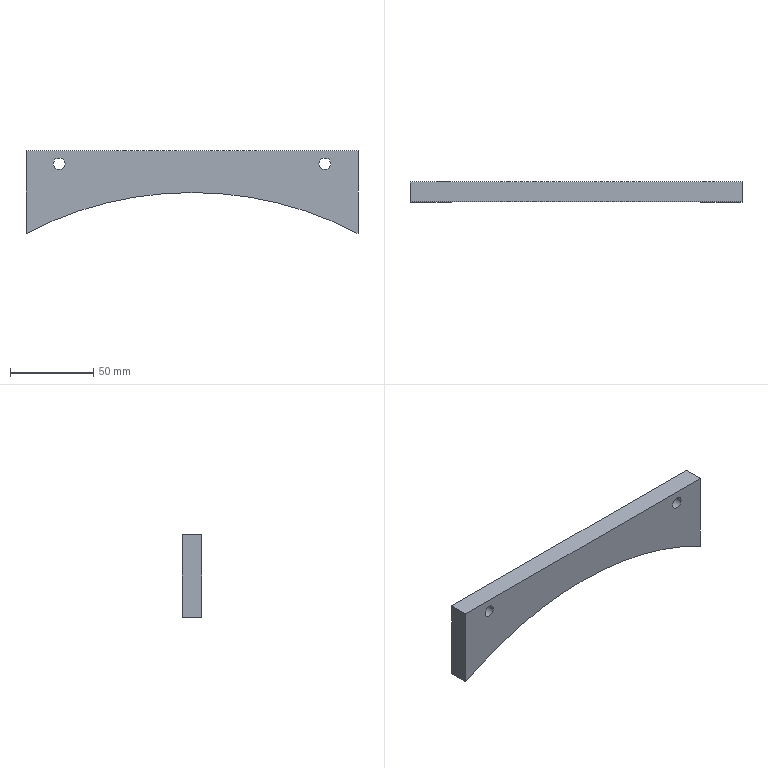Component | SolidWorks | DiscLimitPlate-1 | 1 solid | 10 faces | box 200 x 12 x 50 mm | volume 79126 mm3 | cylinder 5 | plane 5 | commonest cylinder face diameters 7 x4 430 x1
build123d program:
from build123d import *

# Parameters (mm, degrees)
EXTRUDE1_DEPTH = 12
SKETCH2_R      = 3.5
EXTRUDE2_DEPTH = 12


with BuildPart() as part:
    # Sketch1 → Extrude1 (new body)
    with BuildSketch(Plane.XY):
        with BuildLine():
            Line((-100, 0), (-100, -50))
            Line((-100, -50), (100, -50))
            Line((100, -50), (100, 0))
            ThreePointArc((100, 0), (0, -24.671), (-100, 0))
        make_face()
    extrude(amount=EXTRUDE1_DEPTH)

    # Sketch2 → Extrude2 (cut)
    with BuildSketch(Plane.XY.offset(12)):
        with Locations((-80, -42)):
            Circle(SKETCH2_R)
        with Locations((80, -42)):
            Circle(SKETCH2_R)
    extrude(amount=-EXTRUDE2_DEPTH, mode=Mode.SUBTRACT)


solid = part.part

# Placed as in the assembly
solid = solid.moved(Location((-164.784, 440.983, 194.329), (-90, 0, 0)))
STEP:
#1=COLOUR_RGB('',0.7922,0.8196,0.9333);
#2=FILL_AREA_STYLE_COLOUR('',#1);
#3=FILL_AREA_STYLE('',(#2));
#4=SURFACE_STYLE_FILL_AREA(#3);
#5=SURFACE_SIDE_STYLE('',(#4));
#6=SURFACE_STYLE_USAGE(.BOTH.,#5);
#7=PRESENTATION_STYLE_ASSIGNMENT((#6));
#8=CARTESIAN_POINT('',(-3.476,17.362,9.304));
#9=VERTEX_POINT('',#8);
#10=CARTESIAN_POINT('',(-3.2,17.362,9.304));
#11=VERTEX_POINT('',#10);
#12=CARTESIAN_POINT('',(-3.338,17.362,9.304));
#13=DIRECTION('',(0.,1.,0.));
#14=DIRECTION('',(1.,0.,0.));
#15=AXIS2_PLACEMENT_3D('',#12,#13,#14);
#16=CIRCLE('',#15,0.1378);
#17=EDGE_CURVE('',#9,#11,#16,.T.);
#18=ORIENTED_EDGE('',*,*,#17,.F.);
#19=CARTESIAN_POINT('',(-3.476,17.834,9.304));
#20=VERTEX_POINT('',#19);
#21=CARTESIAN_POINT('',(-3.476,17.362,9.304));
#22=DIRECTION('',(0.,1.,0.));
#23=VECTOR('',#22,39.37);
#24=LINE('',#21,#23);
#25=EDGE_CURVE('',#9,#20,#24,.T.);
#26=ORIENTED_EDGE('',*,*,#25,.T.);
#27=CARTESIAN_POINT('',(-3.2,17.834,9.304));
#28=VERTEX_POINT('',#27);
#29=CARTESIAN_POINT('',(-3.338,17.834,9.304));
#30=DIRECTION('',(0.,1.,0.));
#31=DIRECTION('',(1.,0.,0.));
#32=AXIS2_PLACEMENT_3D('',#29,#30,#31);
#33=CIRCLE('',#32,0.1378);
#34=EDGE_CURVE('',#20,#28,#33,.T.);
#35=ORIENTED_EDGE('',*,*,#34,.T.);
#36=CARTESIAN_POINT('',(-3.2,17.362,9.304));
#37=DIRECTION('',(0.,1.,0.));
#38=VECTOR('',#37,39.37);
#39=LINE('',#36,#38);
#40=EDGE_CURVE('',#11,#28,#39,.T.);
#41=ORIENTED_EDGE('',*,*,#40,.F.);
#42=EDGE_LOOP('',(#18,#26,#35,#41));
#43=FACE_OUTER_BOUND('',#42,.T.);
#44=CARTESIAN_POINT('',(-3.338,17.362,9.304));
#45=DIRECTION('',(0.,1.,0.));
#46=DIRECTION('',(1.,0.,0.));
#47=AXIS2_PLACEMENT_3D('',#44,#45,#46);
#48=CYLINDRICAL_SURFACE('',#47,0.1378);
#49=ADVANCED_FACE('',(#43),#48,.F.);
#50=CARTESIAN_POINT('',(-9.775,17.362,9.304));
#51=VERTEX_POINT('',#50);
#52=CARTESIAN_POINT('',(-9.499,17.362,9.304));
#53=VERTEX_POINT('',#52);
#54=CARTESIAN_POINT('',(-9.637,17.362,9.304));
#55=DIRECTION('',(0.,1.,0.));
#56=DIRECTION('',(1.,0.,0.));
#57=AXIS2_PLACEMENT_3D('',#54,#55,#56);
#58=CIRCLE('',#57,0.1378);
#59=EDGE_CURVE('',#51,#53,#58,.T.);
#60=ORIENTED_EDGE('',*,*,#59,.F.);
#61=CARTESIAN_POINT('',(-9.775,17.834,9.304));
#62=VERTEX_POINT('',#61);
#63=CARTESIAN_POINT('',(-9.775,17.362,9.304));
#64=DIRECTION('',(0.,1.,0.));
#65=VECTOR('',#64,39.37);
#66=LINE('',#63,#65);
#67=EDGE_CURVE('',#51,#62,#66,.T.);
#68=ORIENTED_EDGE('',*,*,#67,.T.);
#69=CARTESIAN_POINT('',(-9.499,17.834,9.304));
#70=VERTEX_POINT('',#69);
#71=CARTESIAN_POINT('',(-9.637,17.834,9.304));
#72=DIRECTION('',(0.,1.,0.));
#73=DIRECTION('',(1.,0.,0.));
#74=AXIS2_PLACEMENT_3D('',#71,#72,#73);
#75=CIRCLE('',#74,0.1378);
#76=EDGE_CURVE('',#62,#70,#75,.T.);
#77=ORIENTED_EDGE('',*,*,#76,.T.);
#78=CARTESIAN_POINT('',(-9.499,17.362,9.304));
#79=DIRECTION('',(0.,1.,0.));
#80=VECTOR('',#79,39.37);
#81=LINE('',#78,#80);
#82=EDGE_CURVE('',#53,#70,#81,.T.);
#83=ORIENTED_EDGE('',*,*,#82,.F.);
#84=EDGE_LOOP('',(#60,#68,#77,#83));
#85=FACE_OUTER_BOUND('',#84,.T.);
#86=CARTESIAN_POINT('',(-9.637,17.362,9.304));
#87=DIRECTION('',(0.,1.,0.));
#88=DIRECTION('',(1.,0.,0.));
#89=AXIS2_PLACEMENT_3D('',#86,#87,#88);
#90=CYLINDRICAL_SURFACE('',#89,0.1378);
#91=ADVANCED_FACE('',(#85),#90,.F.);
#92=CARTESIAN_POINT('',(-2.551,17.362,7.651));
#93=VERTEX_POINT('',#92);
#94=CARTESIAN_POINT('',(-10.425,17.362,7.651));
#95=VERTEX_POINT('',#94);
#96=CARTESIAN_POINT('',(-6.488,17.362,0.1575));
#97=DIRECTION('',(0.,-1.,0.));
#98=DIRECTION('',(-1.,0.,0.));
#99=AXIS2_PLACEMENT_3D('',#96,#97,#98);
#100=CIRCLE('',#99,8.465);
#101=EDGE_CURVE('',#93,#95,#100,.T.);
#102=ORIENTED_EDGE('',*,*,#101,.T.);
#103=CARTESIAN_POINT('',(-10.425,17.834,7.651));
#104=VERTEX_POINT('',#103);
#105=CARTESIAN_POINT('',(-10.425,17.834,7.651));
#106=DIRECTION('',(0.,-1.,0.));
#107=VECTOR('',#106,39.37);
#108=LINE('',#105,#107);
#109=EDGE_CURVE('',#104,#95,#108,.T.);
#110=ORIENTED_EDGE('',*,*,#109,.F.);
#111=CARTESIAN_POINT('',(-2.551,17.834,7.651));
#112=VERTEX_POINT('',#111);
#113=CARTESIAN_POINT('',(-6.488,17.834,0.1575));
#114=DIRECTION('',(0.,-1.,0.));
#115=DIRECTION('',(-1.,0.,0.));
#116=AXIS2_PLACEMENT_3D('',#113,#114,#115);
#117=CIRCLE('',#116,8.465);
#118=EDGE_CURVE('',#112,#104,#117,.T.);
#119=ORIENTED_EDGE('',*,*,#118,.F.);
#120=CARTESIAN_POINT('',(-2.551,17.834,7.651));
#121=DIRECTION('',(0.,-1.,0.));
#122=VECTOR('',#121,39.37);
#123=LINE('',#120,#122);
#124=EDGE_CURVE('',#112,#93,#123,.T.);
#125=ORIENTED_EDGE('',*,*,#124,.T.);
#126=EDGE_LOOP('',(#102,#110,#119,#125));
#127=FACE_OUTER_BOUND('',#126,.T.);
#128=CARTESIAN_POINT('',(-6.488,17.834,0.1575));
#129=DIRECTION('',(0.,-1.,0.));
#130=DIRECTION('',(-1.,0.,0.));
#131=AXIS2_PLACEMENT_3D('',#128,#129,#130);
#132=CYLINDRICAL_SURFACE('',#131,8.465);
#133=ADVANCED_FACE('',(#127),#132,.F.);
#134=CARTESIAN_POINT('',(-10.425,17.362,9.619));
#135=VERTEX_POINT('',#134);
#136=CARTESIAN_POINT('',(-10.425,17.362,7.651));
#137=DIRECTION('',(0.,0.,1.));
#138=VECTOR('',#137,39.37);
#139=LINE('',#136,#138);
#140=EDGE_CURVE('',#95,#135,#139,.T.);
#141=ORIENTED_EDGE('',*,*,#140,.T.);
#142=CARTESIAN_POINT('',(-10.425,17.834,9.619));
#143=VERTEX_POINT('',#142);
#144=CARTESIAN_POINT('',(-10.425,17.834,9.619));
#145=DIRECTION('',(0.,-1.,0.));
#146=VECTOR('',#145,39.37);
#147=LINE('',#144,#146);
#148=EDGE_CURVE('',#143,#135,#147,.T.);
#149=ORIENTED_EDGE('',*,*,#148,.F.);
#150=CARTESIAN_POINT('',(-10.425,17.834,7.651));
#151=DIRECTION('',(0.,0.,1.));
#152=VECTOR('',#151,39.37);
#153=LINE('',#150,#152);
#154=EDGE_CURVE('',#104,#143,#153,.T.);
#155=ORIENTED_EDGE('',*,*,#154,.F.);
#156=ORIENTED_EDGE('',*,*,#109,.T.);
#157=EDGE_LOOP('',(#141,#149,#155,#156));
#158=FACE_OUTER_BOUND('',#157,.T.);
#159=CARTESIAN_POINT('',(-10.425,17.834,7.651));
#160=DIRECTION('',(1.,0.,0.));
#161=DIRECTION('',(0.,-1.,0.));
#162=AXIS2_PLACEMENT_3D('',#159,#160,#161);
#163=PLANE('',#162);
#164=ADVANCED_FACE('',(#158),#163,.F.);
#165=CARTESIAN_POINT('',(-2.551,17.362,9.619));
#166=VERTEX_POINT('',#165);
#167=CARTESIAN_POINT('',(-10.425,17.362,9.619));
#168=DIRECTION('',(1.,0.,0.));
#169=VECTOR('',#168,39.37);
#170=LINE('',#167,#169);
#171=EDGE_CURVE('',#135,#166,#170,.T.);
#172=ORIENTED_EDGE('',*,*,#171,.T.);
#173=CARTESIAN_POINT('',(-2.551,17.834,9.619));
#174=VERTEX_POINT('',#173);
#175=CARTESIAN_POINT('',(-2.551,17.834,9.619));
#176=DIRECTION('',(0.,-1.,0.));
#177=VECTOR('',#176,39.37);
#178=LINE('',#175,#177);
#179=EDGE_CURVE('',#174,#166,#178,.T.);
#180=ORIENTED_EDGE('',*,*,#179,.F.);
#181=CARTESIAN_POINT('',(-10.425,17.834,9.619));
#182=DIRECTION('',(1.,0.,0.));
#183=VECTOR('',#182,39.37);
#184=LINE('',#181,#183);
#185=EDGE_CURVE('',#143,#174,#184,.T.);
#186=ORIENTED_EDGE('',*,*,#185,.F.);
#187=ORIENTED_EDGE('',*,*,#148,.T.);
#188=EDGE_LOOP('',(#172,#180,#186,#187));
#189=FACE_OUTER_BOUND('',#188,.T.);
#190=CARTESIAN_POINT('',(-10.425,17.834,9.619));
#191=DIRECTION('',(0.,0.,-1.));
#192=DIRECTION('',(0.,1.,0.));
#193=AXIS2_PLACEMENT_3D('',#190,#191,#192);
#194=PLANE('',#193);
#195=ADVANCED_FACE('',(#189),#194,.F.);
#196=CARTESIAN_POINT('',(-2.551,17.362,7.651));
#197=DIRECTION('',(0.,0.,-1.));
#198=VECTOR('',#197,39.37);
#199=LINE('',#196,#198);
#200=EDGE_CURVE('',#166,#93,#199,.T.);
#201=ORIENTED_EDGE('',*,*,#200,.T.);
#202=ORIENTED_EDGE('',*,*,#124,.F.);
#203=CARTESIAN_POINT('',(-2.551,17.834,7.651));
#204=DIRECTION('',(0.,0.,-1.));
#205=VECTOR('',#204,39.37);
#206=LINE('',#203,#205);
#207=EDGE_CURVE('',#174,#112,#206,.T.);
#208=ORIENTED_EDGE('',*,*,#207,.F.);
#209=ORIENTED_EDGE('',*,*,#179,.T.);
#210=EDGE_LOOP('',(#201,#202,#208,#209));
#211=FACE_OUTER_BOUND('',#210,.T.);
#212=CARTESIAN_POINT('',(-2.551,17.834,7.651));
#213=DIRECTION('',(-1.,0.,0.));
#214=DIRECTION('',(0.,1.,0.));
#215=AXIS2_PLACEMENT_3D('',#212,#213,#214);
#216=PLANE('',#215);
#217=ADVANCED_FACE('',(#211),#216,.F.);
#218=CARTESIAN_POINT('',(-3.338,17.834,9.304));
#219=DIRECTION('',(0.,1.,0.));
#220=DIRECTION('',(1.,0.,0.));
#221=AXIS2_PLACEMENT_3D('',#218,#219,#220);
#222=CIRCLE('',#221,0.1378);
#223=EDGE_CURVE('',#28,#20,#222,.T.);
#224=ORIENTED_EDGE('',*,*,#223,.F.);
#225=ORIENTED_EDGE('',*,*,#34,.F.);
#226=EDGE_LOOP('',(#224,#225));
#227=FACE_BOUND('',#226,.T.);
#228=CARTESIAN_POINT('',(-9.637,17.834,9.304));
#229=DIRECTION('',(0.,1.,0.));
#230=DIRECTION('',(1.,0.,0.));
#231=AXIS2_PLACEMENT_3D('',#228,#229,#230);
#232=CIRCLE('',#231,0.1378);
#233=EDGE_CURVE('',#70,#62,#232,.T.);
#234=ORIENTED_EDGE('',*,*,#233,.F.);
#235=ORIENTED_EDGE('',*,*,#76,.F.);
#236=EDGE_LOOP('',(#234,#235));
#237=FACE_BOUND('',#236,.T.);
#238=ORIENTED_EDGE('',*,*,#118,.T.);
#239=ORIENTED_EDGE('',*,*,#154,.T.);
#240=ORIENTED_EDGE('',*,*,#185,.T.);
#241=ORIENTED_EDGE('',*,*,#207,.T.);
#242=EDGE_LOOP('',(#238,#239,#240,#241));
#243=FACE_OUTER_BOUND('',#242,.T.);
#244=CARTESIAN_POINT('',(-6.488,17.834,0.1575));
#245=DIRECTION('',(0.,-1.,0.));
#246=DIRECTION('',(-1.,0.,0.));
#247=AXIS2_PLACEMENT_3D('',#244,#245,#246);
#248=PLANE('',#247);
#249=ADVANCED_FACE('',(#227,#237,#243),#248,.F.);
#250=CARTESIAN_POINT('',(-3.338,17.362,9.304));
#251=DIRECTION('',(0.,1.,0.));
#252=DIRECTION('',(1.,0.,0.));
#253=AXIS2_PLACEMENT_3D('',#250,#251,#252);
#254=CIRCLE('',#253,0.1378);
#255=EDGE_CURVE('',#11,#9,#254,.T.);
#256=ORIENTED_EDGE('',*,*,#255,.T.);
#257=ORIENTED_EDGE('',*,*,#17,.T.);
#258=EDGE_LOOP('',(#256,#257));
#259=FACE_BOUND('',#258,.T.);
#260=CARTESIAN_POINT('',(-9.637,17.362,9.304));
#261=DIRECTION('',(0.,1.,0.));
#262=DIRECTION('',(1.,0.,0.));
#263=AXIS2_PLACEMENT_3D('',#260,#261,#262);
#264=CIRCLE('',#263,0.1378);
#265=EDGE_CURVE('',#53,#51,#264,.T.);
#266=ORIENTED_EDGE('',*,*,#265,.T.);
#267=ORIENTED_EDGE('',*,*,#59,.T.);
#268=EDGE_LOOP('',(#266,#267));
#269=FACE_BOUND('',#268,.T.);
#270=ORIENTED_EDGE('',*,*,#101,.F.);
#271=ORIENTED_EDGE('',*,*,#200,.F.);
#272=ORIENTED_EDGE('',*,*,#171,.F.);
#273=ORIENTED_EDGE('',*,*,#140,.F.);
#274=EDGE_LOOP('',(#270,#271,#272,#273));
#275=FACE_OUTER_BOUND('',#274,.T.);
#276=CARTESIAN_POINT('',(-6.488,17.362,0.1575));
#277=DIRECTION('',(0.,-1.,0.));
#278=DIRECTION('',(-1.,0.,0.));
#279=AXIS2_PLACEMENT_3D('',#276,#277,#278);
#280=PLANE('',#279);
#281=ADVANCED_FACE('',(#259,#269,#275),#280,.T.);
#282=ORIENTED_EDGE('',*,*,#67,.F.);
#283=ORIENTED_EDGE('',*,*,#265,.F.);
#284=ORIENTED_EDGE('',*,*,#82,.T.);
#285=ORIENTED_EDGE('',*,*,#233,.T.);
#286=EDGE_LOOP('',(#282,#283,#284,#285));
#287=FACE_OUTER_BOUND('',#286,.T.);
#288=CARTESIAN_POINT('',(-9.637,17.362,9.304));
#289=DIRECTION('',(0.,1.,0.));
#290=DIRECTION('',(1.,0.,0.));
#291=AXIS2_PLACEMENT_3D('',#288,#289,#290);
#292=CYLINDRICAL_SURFACE('',#291,0.1378);
#293=ADVANCED_FACE('',(#287),#292,.F.);
#294=ORIENTED_EDGE('',*,*,#25,.F.);
#295=ORIENTED_EDGE('',*,*,#255,.F.);
#296=ORIENTED_EDGE('',*,*,#40,.T.);
#297=ORIENTED_EDGE('',*,*,#223,.T.);
#298=EDGE_LOOP('',(#294,#295,#296,#297));
#299=FACE_OUTER_BOUND('',#298,.T.);
#300=CARTESIAN_POINT('',(-3.338,17.362,9.304));
#301=DIRECTION('',(0.,1.,0.));
#302=DIRECTION('',(1.,0.,0.));
#303=AXIS2_PLACEMENT_3D('',#300,#301,#302);
#304=CYLINDRICAL_SURFACE('',#303,0.1378);
#305=ADVANCED_FACE('',(#299),#304,.F.);
#306=CLOSED_SHELL('',(#49,#91,#133,#164,#195,#217,#249,#281,#293,#305));
#307=MANIFOLD_SOLID_BREP('',#306);
#308=STYLED_ITEM('',(#7),#307);
#309=PRESENTATION_LAYER_ASSIGNMENT('','',(#308));
#310=CARTESIAN_POINT('',(0.,0.,0.));
#311=DIRECTION('',(0.,0.,1.));
#312=DIRECTION('',(1.,0.,0.));
#313=AXIS2_PLACEMENT_3D('',#310,#311,#312);
#314=(LENGTH_UNIT()NAMED_UNIT(*)SI_UNIT($,.METRE.));
#315=LENGTH_MEASURE_WITH_UNIT(LENGTH_MEASURE(0.0254),#314);
#316=DIMENSIONAL_EXPONENTS(1.,0.,0.,0.,0.,0.,0.);
#317=(CONVERSION_BASED_UNIT('',#315)LENGTH_UNIT()NAMED_UNIT(#316));
#318=UNCERTAINTY_MEASURE_WITH_UNIT(LENGTH_MEASURE(0.00001),#317,'','');
#319=(NAMED_UNIT(*)PLANE_ANGLE_UNIT()SI_UNIT($,.RADIAN.));
#320=(NAMED_UNIT(*)SI_UNIT($,.STERADIAN.)SOLID_ANGLE_UNIT());
#321=(GEOMETRIC_REPRESENTATION_CONTEXT(3)GLOBAL_UNCERTAINTY_ASSIGNED_CONTEXT((#318))GLOBAL_UNIT_ASSIGNED_CONTEXT((#317,#319,#320))REPRESENTATION_CONTEXT('',''));
#322=ADVANCED_BREP_SHAPE_REPRESENTATION('',(#307,#313),#321);
#323=(LENGTH_UNIT()NAMED_UNIT(*)SI_UNIT($,.METRE.));
#324=LENGTH_MEASURE_WITH_UNIT(LENGTH_MEASURE(0.0254),#323);
#325=DIMENSIONAL_EXPONENTS(1.,0.,0.,0.,0.,0.,0.);
#326=(CONVERSION_BASED_UNIT('',#324)LENGTH_UNIT()NAMED_UNIT(#325));
#327=UNCERTAINTY_MEASURE_WITH_UNIT(LENGTH_MEASURE(0.00001),#326,'','');
#328=(NAMED_UNIT(*)PLANE_ANGLE_UNIT()SI_UNIT($,.RADIAN.));
#329=(NAMED_UNIT(*)SI_UNIT($,.STERADIAN.)SOLID_ANGLE_UNIT());
#330=(GEOMETRIC_REPRESENTATION_CONTEXT(3)GLOBAL_UNCERTAINTY_ASSIGNED_CONTEXT((#327))GLOBAL_UNIT_ASSIGNED_CONTEXT((#326,#328,#329))REPRESENTATION_CONTEXT('',''));
#331=MECHANICAL_DESIGN_GEOMETRIC_PRESENTATION_REPRESENTATION('',(#308),#330);